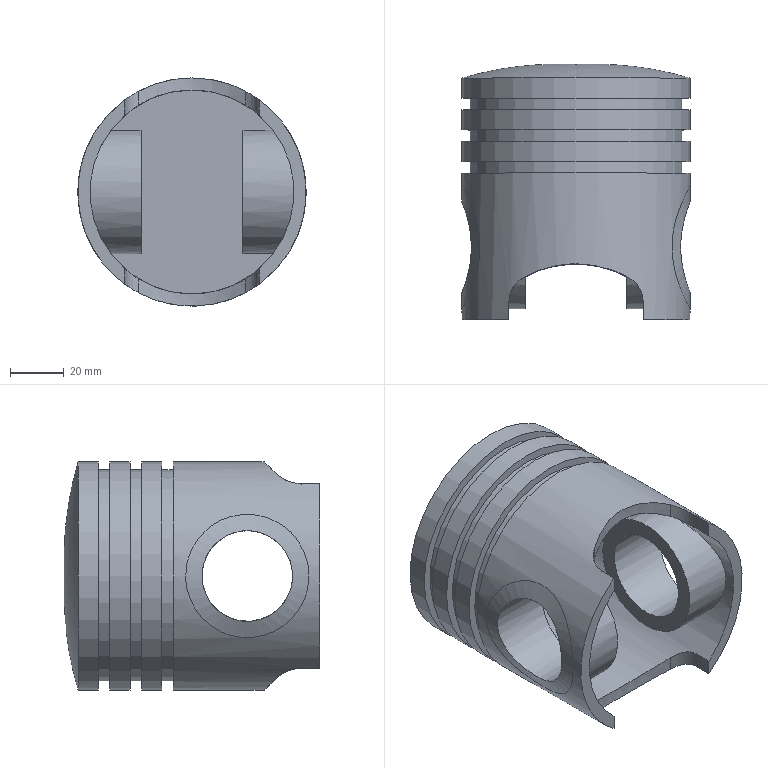Component | NX | 2_PISTON_HEAD | 1 solid | 36 faces | volume 139680 mm3 | cylinder 18 | plane 15 | cone 2 | spline 1 | commonest cylinder face diameters 85 x4 20 x4 79 x3 45.9 x2 33.8 x2 80 x2 76 x1